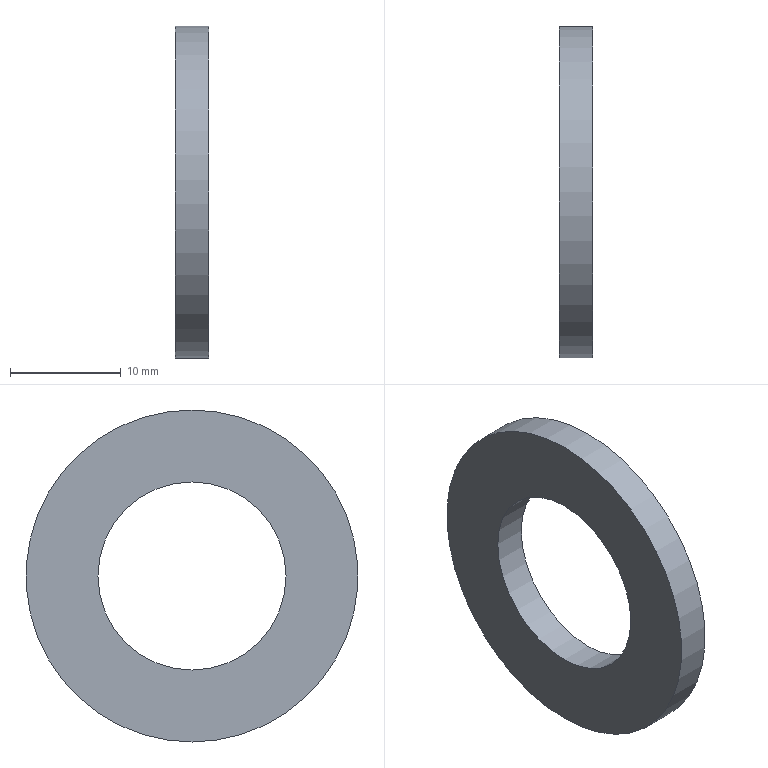Component | NX | GB-T97_1-2002_M16 | 1 solid | 4 faces | box 3 x 30 x 30 mm | volume 1440 mm3 | cylinder 2 | plane 2 | commonest cylinder face diameters 30 x1 17 x1
STEP:
#1=CARTESIAN_POINT('',(0.,0.,0.));
#2=DIRECTION('',(0.,0.,1.));
#3=DIRECTION('',(1.,0.,0.));
#4=AXIS2_PLACEMENT_3D('',#1,#2,#3);
#5=CARTESIAN_POINT('',(-43.,-15.8,148.669));
#6=VERTEX_POINT('',#5);
#7=CARTESIAN_POINT('',(-43.,-15.8,133.669));
#8=DIRECTION('',(-1.,0.,0.));
#9=DIRECTION('',(0.,0.,1.));
#10=AXIS2_PLACEMENT_3D('',#7,#8,#9);
#11=CIRCLE('',#10,15.);
#12=CARTESIAN_POINT('',(-43.,-15.8,133.669));
#13=DIRECTION('',(1.,0.,0.));
#14=DIRECTION('',(0.,0.,-1.));
#15=AXIS2_PLACEMENT_3D('',#12,#13,#14);
#16=CYLINDRICAL_SURFACE('',#15,15.);
#17=CARTESIAN_POINT('',(9.425,0.));
#18=DIRECTION('',(-1.,0.));
#19=VECTOR('',#18,1.);
#20=LINE('',#17,#19);
#21=(GEOMETRIC_REPRESENTATION_CONTEXT(2)PARAMETRIC_REPRESENTATION_CONTEXT()REPRESENTATION_CONTEXT('',''));
#22=DEFINITIONAL_REPRESENTATION('',(#20),#21);
#23=PCURVE('',#16,#22);
#24=CARTESIAN_POINT('',(-43.,-15.8,133.669));
#25=DIRECTION('',(-1.,0.,0.));
#26=DIRECTION('',(0.,0.,1.));
#27=AXIS2_PLACEMENT_3D('',#24,#25,#26);
#28=PLANE('',#27);
#29=CARTESIAN_POINT('',(0.,0.));
#30=DIRECTION('',(1.,0.));
#31=AXIS2_PLACEMENT_2D('',#29,#30);
#32=CIRCLE('',#31,15.);
#33=(GEOMETRIC_REPRESENTATION_CONTEXT(2)PARAMETRIC_REPRESENTATION_CONTEXT()REPRESENTATION_CONTEXT('',''));
#34=DEFINITIONAL_REPRESENTATION('',(#32),#33);
#35=PCURVE('',#28,#34);
#36=SURFACE_CURVE('',#11,(#23,#35),.PCURVE_S1.);
#37=EDGE_CURVE('',#6,#6,#36,.T.);
#38=ORIENTED_EDGE('',*,*,#37,.F.);
#39=CARTESIAN_POINT('',(-40.,-15.8,148.669));
#40=VERTEX_POINT('',#39);
#41=CARTESIAN_POINT('',(-43.,-15.8,148.669));
#42=CARTESIAN_POINT('',(-40.,-15.8,148.669));
#43=B_SPLINE_CURVE_WITH_KNOTS('',1,(#41,#42),.UNSPECIFIED.,.F.,.F.,(2,2),(0.,3.),.PIECEWISE_BEZIER_KNOTS.);
#44=CARTESIAN_POINT('',(9.425,0.));
#45=DIRECTION('',(0.,1.));
#46=VECTOR('',#45,1.);
#47=LINE('',#44,#46);
#48=(GEOMETRIC_REPRESENTATION_CONTEXT(2)PARAMETRIC_REPRESENTATION_CONTEXT()REPRESENTATION_CONTEXT('',''));
#49=DEFINITIONAL_REPRESENTATION('',(#47),#48);
#50=PCURVE('',#16,#49);
#51=CARTESIAN_POINT('',(3.142,0.));
#52=DIRECTION('',(0.,1.));
#53=VECTOR('',#52,1.);
#54=LINE('',#51,#53);
#55=(GEOMETRIC_REPRESENTATION_CONTEXT(2)PARAMETRIC_REPRESENTATION_CONTEXT()REPRESENTATION_CONTEXT('',''));
#56=DEFINITIONAL_REPRESENTATION('',(#54),#55);
#57=PCURVE('',#16,#56);
#58=SEAM_CURVE('',#43,(#50,#57),.PCURVE_S1.);
#59=EDGE_CURVE('',#6,#40,#58,.T.);
#60=ORIENTED_EDGE('',*,*,#59,.T.);
#61=CARTESIAN_POINT('',(-40.,-15.8,133.669));
#62=DIRECTION('',(-1.,0.,0.));
#63=DIRECTION('',(0.,0.,1.));
#64=AXIS2_PLACEMENT_3D('',#61,#62,#63);
#65=CIRCLE('',#64,15.);
#66=CARTESIAN_POINT('',(9.425,3.));
#67=DIRECTION('',(-1.,0.));
#68=VECTOR('',#67,1.);
#69=LINE('',#66,#68);
#70=(GEOMETRIC_REPRESENTATION_CONTEXT(2)PARAMETRIC_REPRESENTATION_CONTEXT()REPRESENTATION_CONTEXT('',''));
#71=DEFINITIONAL_REPRESENTATION('',(#69),#70);
#72=PCURVE('',#16,#71);
#73=CARTESIAN_POINT('',(-40.,-15.8,133.669));
#74=DIRECTION('',(-1.,0.,0.));
#75=DIRECTION('',(0.,0.,1.));
#76=AXIS2_PLACEMENT_3D('',#73,#74,#75);
#77=PLANE('',#76);
#78=CARTESIAN_POINT('',(0.,0.));
#79=DIRECTION('',(1.,0.));
#80=AXIS2_PLACEMENT_2D('',#78,#79);
#81=CIRCLE('',#80,15.);
#82=(GEOMETRIC_REPRESENTATION_CONTEXT(2)PARAMETRIC_REPRESENTATION_CONTEXT()REPRESENTATION_CONTEXT('',''));
#83=DEFINITIONAL_REPRESENTATION('',(#81),#82);
#84=PCURVE('',#77,#83);
#85=SURFACE_CURVE('',#65,(#72,#84),.PCURVE_S1.);
#86=EDGE_CURVE('',#40,#40,#85,.T.);
#87=ORIENTED_EDGE('',*,*,#86,.T.);
#88=ORIENTED_EDGE('',*,*,#59,.F.);
#89=EDGE_LOOP('',(#38,#60,#87,#88));
#90=FACE_BOUND('',#89,.T.);
#91=ADVANCED_FACE('',(#90),#16,.T.);
#92=CARTESIAN_POINT('',(-43.,-15.8,142.169));
#93=VERTEX_POINT('',#92);
#94=CARTESIAN_POINT('',(-43.,-15.8,133.669));
#95=DIRECTION('',(-1.,0.,0.));
#96=DIRECTION('',(0.,0.,1.));
#97=AXIS2_PLACEMENT_3D('',#94,#95,#96);
#98=CIRCLE('',#97,8.5);
#99=CARTESIAN_POINT('',(-43.,-15.8,133.669));
#100=DIRECTION('',(1.,0.,0.));
#101=DIRECTION('',(0.,0.,-1.));
#102=AXIS2_PLACEMENT_3D('',#99,#100,#101);
#103=CYLINDRICAL_SURFACE('',#102,8.5);
#104=CARTESIAN_POINT('',(9.425,0.));
#105=DIRECTION('',(-1.,0.));
#106=VECTOR('',#105,1.);
#107=LINE('',#104,#106);
#108=(GEOMETRIC_REPRESENTATION_CONTEXT(2)PARAMETRIC_REPRESENTATION_CONTEXT()REPRESENTATION_CONTEXT('',''));
#109=DEFINITIONAL_REPRESENTATION('',(#107),#108);
#110=PCURVE('',#103,#109);
#111=CARTESIAN_POINT('',(0.,0.));
#112=DIRECTION('',(1.,0.));
#113=AXIS2_PLACEMENT_2D('',#111,#112);
#114=CIRCLE('',#113,8.5);
#115=(GEOMETRIC_REPRESENTATION_CONTEXT(2)PARAMETRIC_REPRESENTATION_CONTEXT()REPRESENTATION_CONTEXT('',''));
#116=DEFINITIONAL_REPRESENTATION('',(#114),#115);
#117=PCURVE('',#28,#116);
#118=SURFACE_CURVE('',#98,(#110,#117),.PCURVE_S1.);
#119=EDGE_CURVE('',#93,#93,#118,.T.);
#120=ORIENTED_EDGE('',*,*,#119,.F.);
#121=CARTESIAN_POINT('',(-40.,-15.8,142.169));
#122=VERTEX_POINT('',#121);
#123=CARTESIAN_POINT('',(-43.,-15.8,142.169));
#124=CARTESIAN_POINT('',(-40.,-15.8,142.169));
#125=B_SPLINE_CURVE_WITH_KNOTS('',1,(#123,#124),.UNSPECIFIED.,.F.,.F.,(2,2),(0.,3.),.PIECEWISE_BEZIER_KNOTS.);
#126=CARTESIAN_POINT('',(9.425,0.));
#127=DIRECTION('',(0.,1.));
#128=VECTOR('',#127,1.);
#129=LINE('',#126,#128);
#130=(GEOMETRIC_REPRESENTATION_CONTEXT(2)PARAMETRIC_REPRESENTATION_CONTEXT()REPRESENTATION_CONTEXT('',''));
#131=DEFINITIONAL_REPRESENTATION('',(#129),#130);
#132=PCURVE('',#103,#131);
#133=CARTESIAN_POINT('',(3.142,0.));
#134=DIRECTION('',(0.,1.));
#135=VECTOR('',#134,1.);
#136=LINE('',#133,#135);
#137=(GEOMETRIC_REPRESENTATION_CONTEXT(2)PARAMETRIC_REPRESENTATION_CONTEXT()REPRESENTATION_CONTEXT('',''));
#138=DEFINITIONAL_REPRESENTATION('',(#136),#137);
#139=PCURVE('',#103,#138);
#140=SEAM_CURVE('',#125,(#132,#139),.PCURVE_S1.);
#141=EDGE_CURVE('',#93,#122,#140,.T.);
#142=ORIENTED_EDGE('',*,*,#141,.T.);
#143=CARTESIAN_POINT('',(-40.,-15.8,133.669));
#144=DIRECTION('',(-1.,0.,0.));
#145=DIRECTION('',(0.,0.,1.));
#146=AXIS2_PLACEMENT_3D('',#143,#144,#145);
#147=CIRCLE('',#146,8.5);
#148=CARTESIAN_POINT('',(9.425,3.));
#149=DIRECTION('',(-1.,0.));
#150=VECTOR('',#149,1.);
#151=LINE('',#148,#150);
#152=(GEOMETRIC_REPRESENTATION_CONTEXT(2)PARAMETRIC_REPRESENTATION_CONTEXT()REPRESENTATION_CONTEXT('',''));
#153=DEFINITIONAL_REPRESENTATION('',(#151),#152);
#154=PCURVE('',#103,#153);
#155=CARTESIAN_POINT('',(0.,0.));
#156=DIRECTION('',(1.,0.));
#157=AXIS2_PLACEMENT_2D('',#155,#156);
#158=CIRCLE('',#157,8.5);
#159=(GEOMETRIC_REPRESENTATION_CONTEXT(2)PARAMETRIC_REPRESENTATION_CONTEXT()REPRESENTATION_CONTEXT('',''));
#160=DEFINITIONAL_REPRESENTATION('',(#158),#159);
#161=PCURVE('',#77,#160);
#162=SURFACE_CURVE('',#147,(#154,#161),.PCURVE_S1.);
#163=EDGE_CURVE('',#122,#122,#162,.T.);
#164=ORIENTED_EDGE('',*,*,#163,.T.);
#165=ORIENTED_EDGE('',*,*,#141,.F.);
#166=EDGE_LOOP('',(#120,#142,#164,#165));
#167=FACE_BOUND('',#166,.F.);
#168=ADVANCED_FACE('',(#167),#103,.F.);
#169=ORIENTED_EDGE('',*,*,#37,.T.);
#170=EDGE_LOOP('',(#169));
#171=FACE_BOUND('',#170,.T.);
#172=ORIENTED_EDGE('',*,*,#119,.F.);
#173=EDGE_LOOP('',(#172));
#174=FACE_BOUND('',#173,.T.);
#175=ADVANCED_FACE('',(#171,#174),#28,.T.);
#176=ORIENTED_EDGE('',*,*,#86,.F.);
#177=EDGE_LOOP('',(#176));
#178=FACE_BOUND('',#177,.T.);
#179=ORIENTED_EDGE('',*,*,#163,.T.);
#180=EDGE_LOOP('',(#179));
#181=FACE_BOUND('',#180,.T.);
#182=ADVANCED_FACE('',(#178,#181),#77,.F.);
#183=CLOSED_SHELL('',(#91,#168,#175,#182));
#184=MANIFOLD_SOLID_BREP('',#183);
#185=(LENGTH_UNIT()NAMED_UNIT(*)SI_UNIT(.MILLI.,.METRE.));
#186=UNCERTAINTY_MEASURE_WITH_UNIT(LENGTH_MEASURE(0.00001),#185,'','');
#187=(NAMED_UNIT(*)PLANE_ANGLE_UNIT()SI_UNIT($,.RADIAN.));
#188=(NAMED_UNIT(*)SI_UNIT($,.STERADIAN.)SOLID_ANGLE_UNIT());
#189=(GEOMETRIC_REPRESENTATION_CONTEXT(3)GLOBAL_UNCERTAINTY_ASSIGNED_CONTEXT((#186))GLOBAL_UNIT_ASSIGNED_CONTEXT((#185,#187,#188))REPRESENTATION_CONTEXT('',''));
#190=ADVANCED_BREP_SHAPE_REPRESENTATION('',(#4,#184),#189);